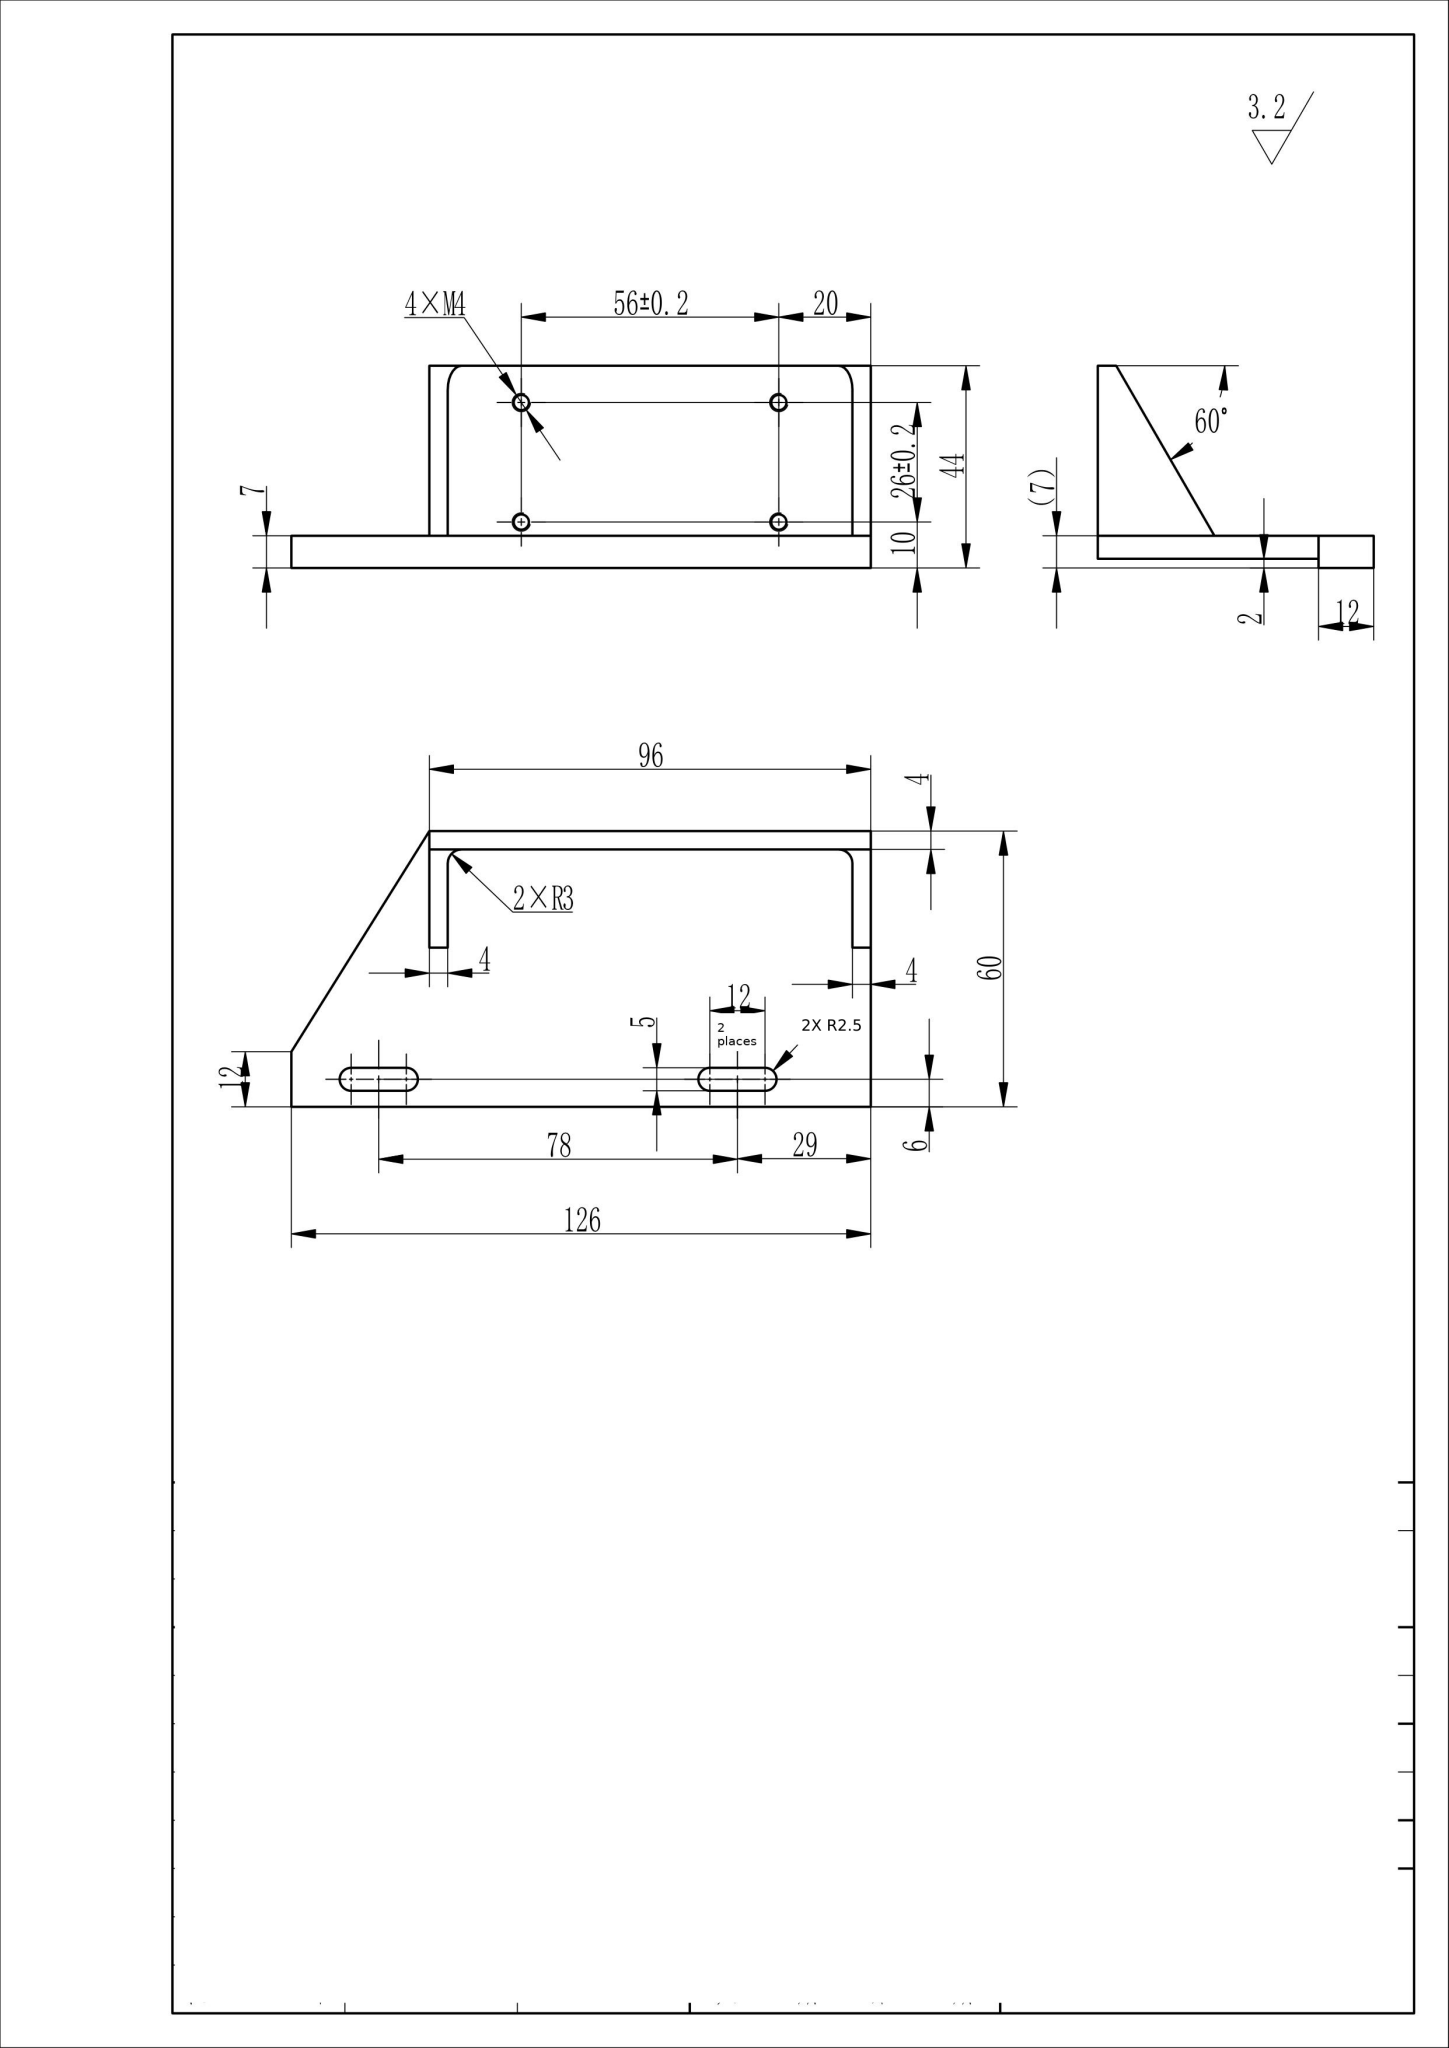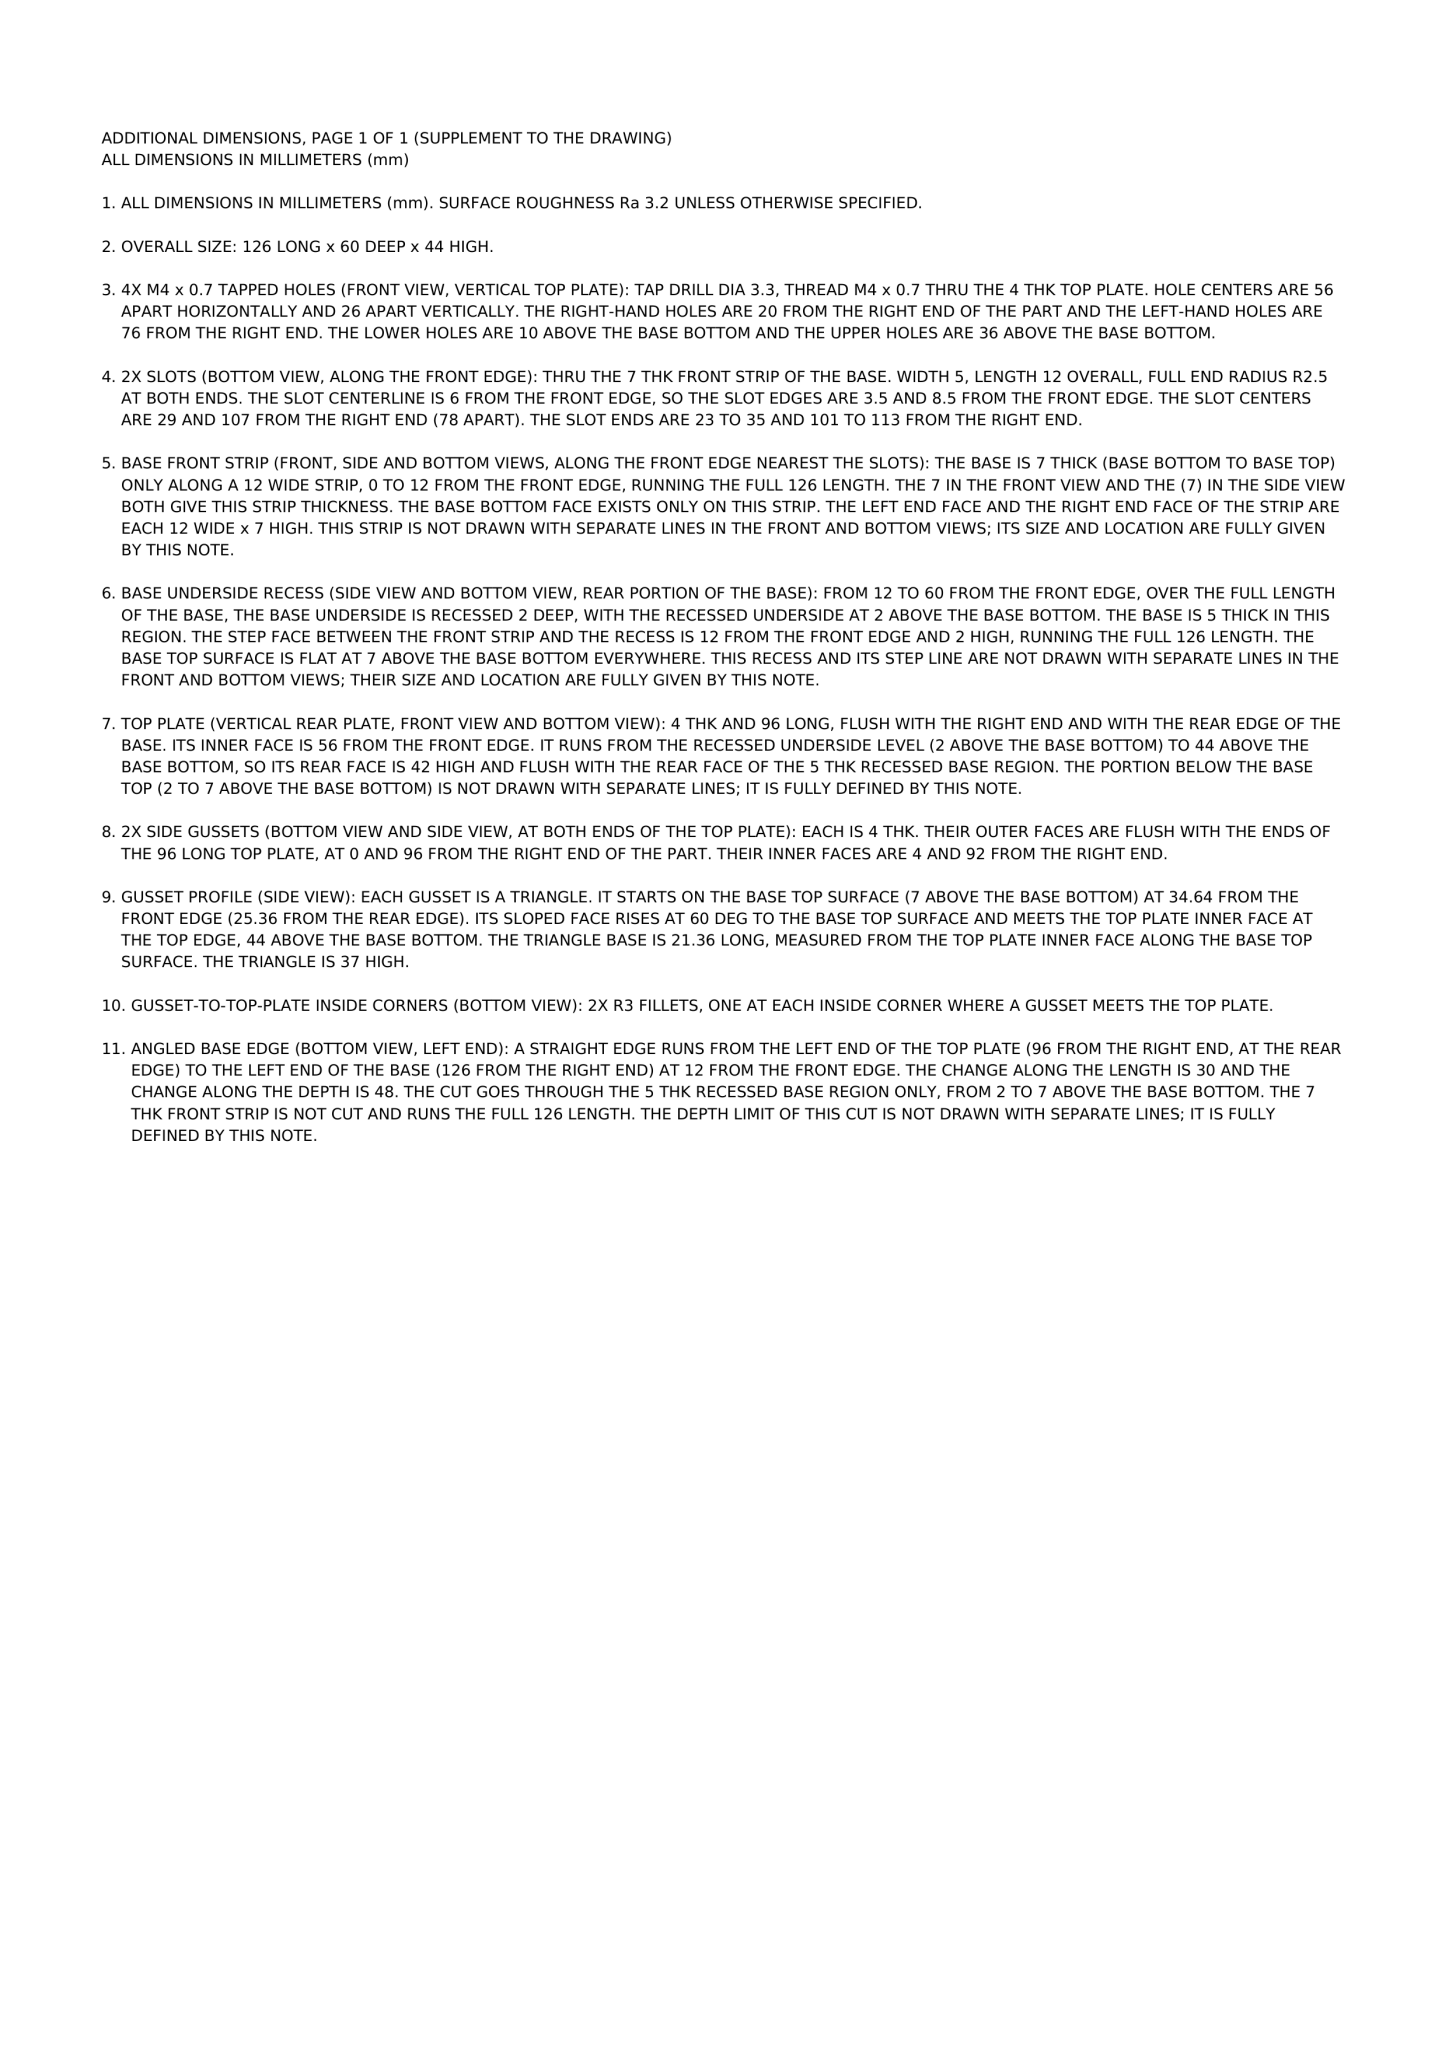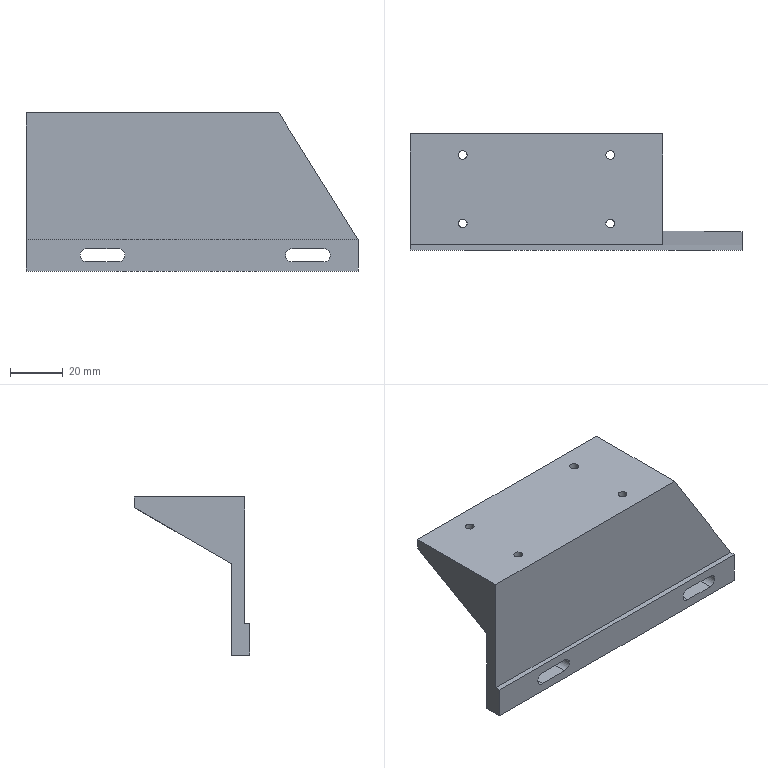Part | NX | mm | 1 solid | 30 faces | box 126 x 44 x 60 mm | volume 53480 mm3 | plane 20 | cylinder 10 | commonest cylinder face diameters 5 x4 3.3 x4 6 x2